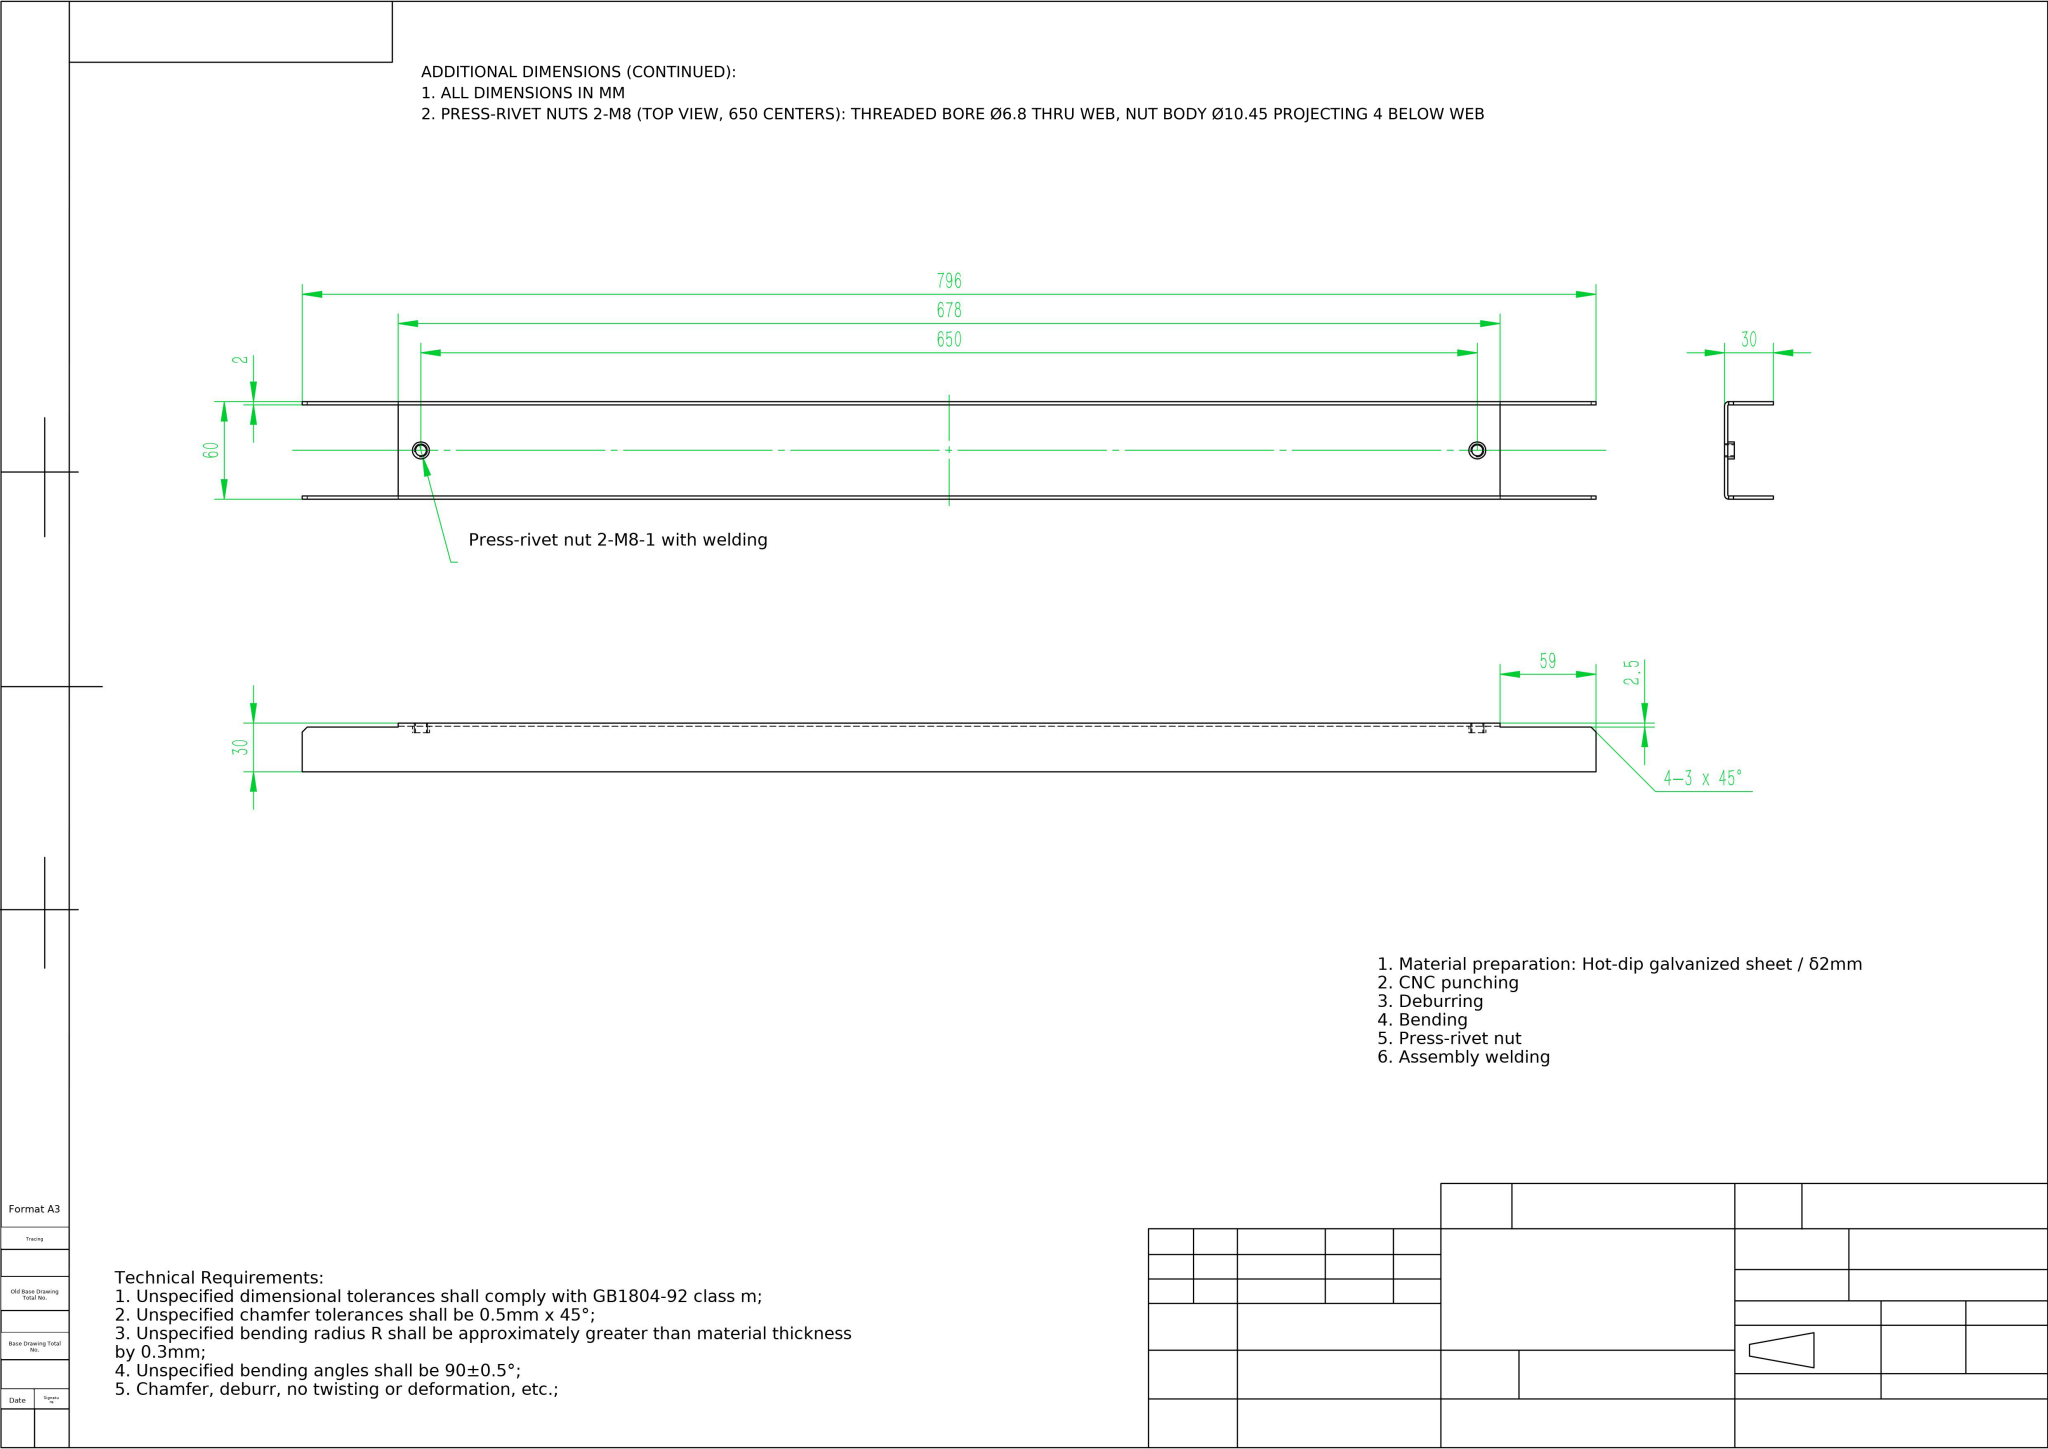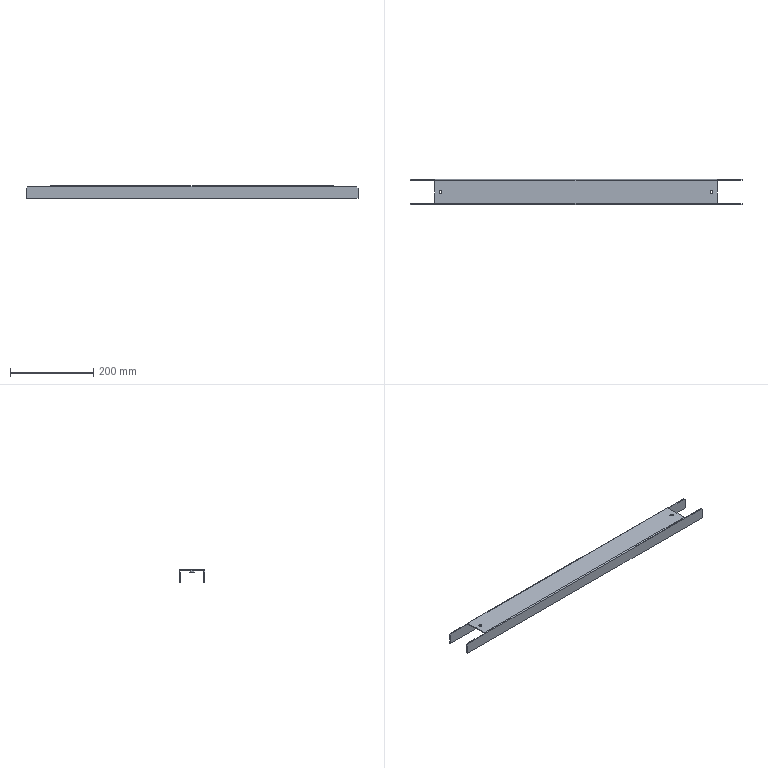Part | NX | mm | 1 solid | 38 faces | box 796 x 60 x 30 mm | volume 168744 mm3 | plane 26 | cylinder 12 | commonest cylinder face diameters 6.8 x4 10.45 x4 5 x2 1 x2